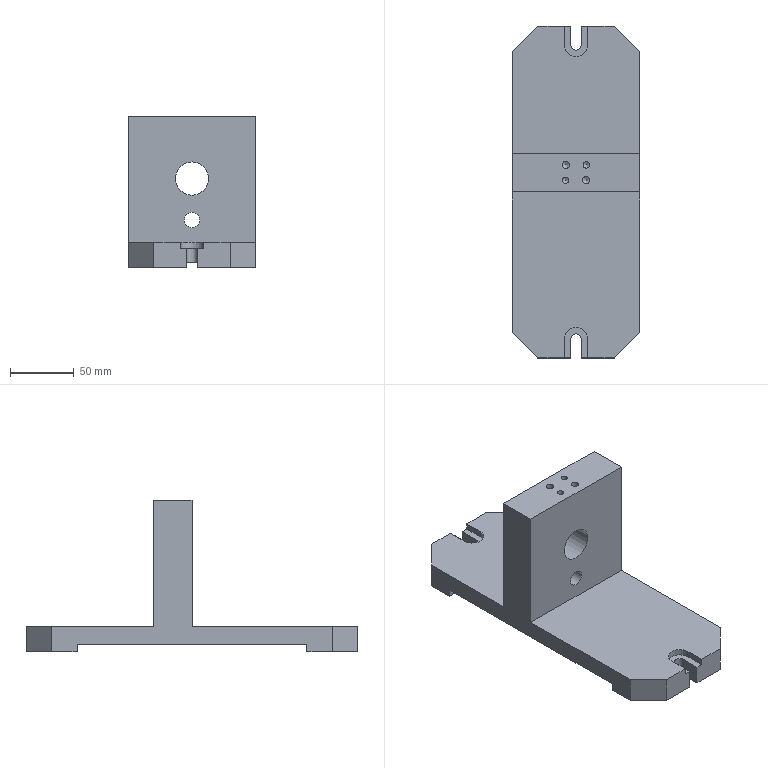Component | NX | FIXTURE_BODY | 1 solid | 58 faces | volume 662761 mm3 | plane 34 | cylinder 15 | cone 9 | commonest cylinder face diameters 1.886 x3 8 x2 5.795 x2 5 x2 18 x2 2.874 x2 12 x1 26 x1